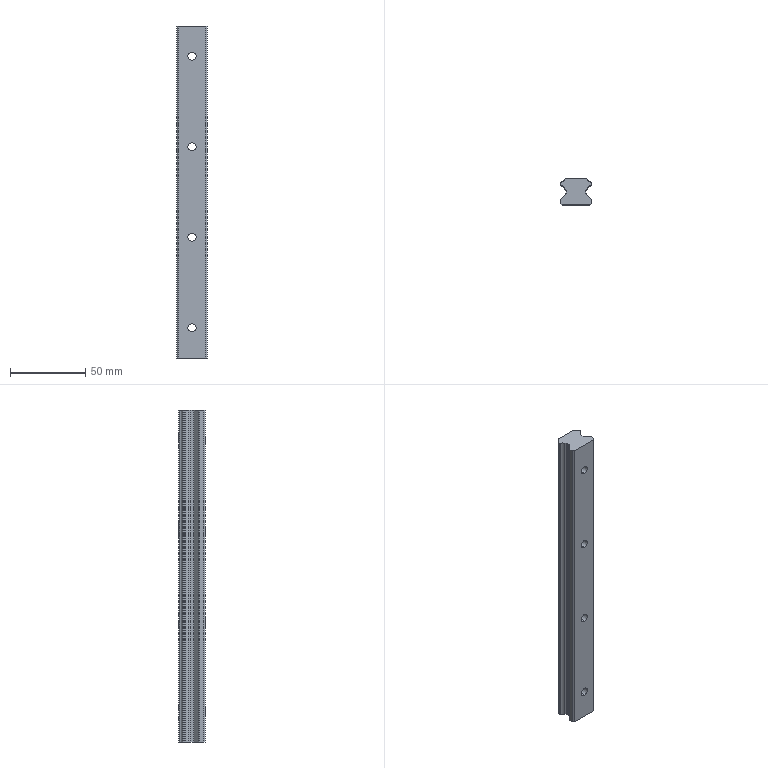Component | SolidWorks | HZ022-HGH-20CAGuideRail-1 | 1 solid | 64 faces | box 20 x 17.5 x 220 mm | volume 62847 mm3 | cylinder 38 | plane 26 | commonest cylinder face diameters 1 x12 5.5 x8 10 x8 2 x6 4.06 x4 | material 45
build123d program:
from build123d import *

# Parameters (mm, degrees)
EXTRUDE1_DEPTH                                       = 220
HOLE_SIZE_ACCORDING_TO_HEXAGON_SOCKET_HE_D           = 5.5
HOLE_SIZE_ACCORDING_TO_HEXAGON_SOCKET_HE_CBORE_D     = 10
HOLE_SIZE_ACCORDING_TO_HEXAGON_SOCKET_HE_CBORE_DEPTH = 5.7
LPATTERN1_COUNT                                      = 4
LPATTERN1_PITCH                                      = 60


with BuildPart() as part:
    # Sketch1 → Extrude1 (new body)
    with BuildSketch(Plane.XY):
        with BuildLine():
            Line((7.648, -0.417), (7.231, 0))
            Line((7.231, 0), (-7.231, 0))
            Line((-7.231, 0), (-7.648, -0.417))
            ThreePointArc((-7.648, -0.417), (-7.736, -0.5369), (-7.785, -0.6776))
            ThreePointArc((-7.785, -0.6776), (-8.345, -1.736), (-9.403, -2.295))
            ThreePointArc((-9.403, -2.295), (-9.543, -2.344), (-9.663, -2.433))
            Line((-9.663, -2.433), (-9.854, -2.623))
            ThreePointArc((-9.854, -2.623), (-9.962, -2.785), (-10, -2.976))
            Line((-10, -2.976), (-10, -4.034))
            ThreePointArc((-10, -4.034), (-9.962, -4.225), (-9.854, -4.387))
            Line((-9.854, -4.387), (-9.675, -4.565))
            ThreePointArc((-9.675, -4.565), (-9.554, -4.654), (-9.412, -4.704))
            ThreePointArc((-9.412, -4.704), (-8.345, -5.265), (-7.784, -6.332))
            ThreePointArc((-7.784, -6.332), (-7.735, -6.474), (-7.645, -6.595))
            Line((-7.645, -6.595), (-6.893, -7.348))
            ThreePointArc((-6.893, -7.348), (-6.676, -7.672), (-6.6, -8.055))
            Line((-6.6, -8.055), (-6.6, -9.615))
            ThreePointArc((-6.6, -9.615), (-6.676, -9.998), (-6.893, -10.322))
            Line((-6.893, -10.322), (-9.707, -13.136))
            ThreePointArc((-9.707, -13.136), (-9.924, -13.461), (-10, -13.843))
            Line((-10, -13.843), (-10, -16.5))
            Line((-10, -16.5), (-9, -17.5))
            Line((-9, -17.5), (9, -17.5))
            Line((9, -17.5), (10, -16.5))
            Line((10, -16.5), (10, -13.843))
            ThreePointArc((10, -13.843), (9.924, -13.461), (9.707, -13.136))
            Line((9.707, -13.136), (6.893, -10.322))
            ThreePointArc((6.893, -10.322), (6.676, -9.998), (6.6, -9.615))
            Line((6.6, -9.615), (6.6, -8.055))
            ThreePointArc((6.6, -8.055), (6.676, -7.672), (6.893, -7.348))
            Line((6.893, -7.348), (7.645, -6.595))
            ThreePointArc((7.645, -6.595), (7.735, -6.474), (7.784, -6.332))
            ThreePointArc((7.784, -6.332), (8.345, -5.265), (9.412, -4.704))
            ThreePointArc((9.412, -4.704), (9.554, -4.654), (9.675, -4.565))
            Line((9.675, -4.565), (9.854, -4.387))
            ThreePointArc((9.854, -4.387), (9.962, -4.225), (10, -4.034))
            Line((10, -4.034), (10, -2.976))
            ThreePointArc((10, -2.976), (9.962, -2.785), (9.854, -2.623))
            Line((9.854, -2.623), (9.663, -2.433))
            ThreePointArc((9.663, -2.433), (9.543, -2.344), (9.403, -2.295))
            ThreePointArc((9.403, -2.295), (8.345, -1.736), (7.785, -0.6776))
            ThreePointArc((7.785, -0.6776), (7.736, -0.5369), (7.648, -0.417))
        make_face()
    extrude(amount=EXTRUDE1_DEPTH)

    # Hole Size according to Hexagon Socket He (through all)
    with Locations(Plane(origin=(0, 0, 0), x_dir=(-1, 0, 0), z_dir=(0, 1, 0))):
        with Locations((0, 20)):
            hole_size_according_to_hexagon_socket_he = CounterBoreHole(HOLE_SIZE_ACCORDING_TO_HEXAGON_SOCKET_HE_D / 2, HOLE_SIZE_ACCORDING_TO_HEXAGON_SOCKET_HE_CBORE_D / 2, HOLE_SIZE_ACCORDING_TO_HEXAGON_SOCKET_HE_CBORE_DEPTH)

    # LPattern1: Hole Size according to Hexagon Socket He ×4
    with Locations(*[(0, 0, i * LPATTERN1_PITCH) for i in range(1, LPATTERN1_COUNT)]):
        add(hole_size_according_to_hexagon_socket_he, mode=Mode.SUBTRACT)


solid = part.part

# Placed as in the assembly
solid = solid.moved(Location((153.744, 32.152, 730), (0, 0, 0)))